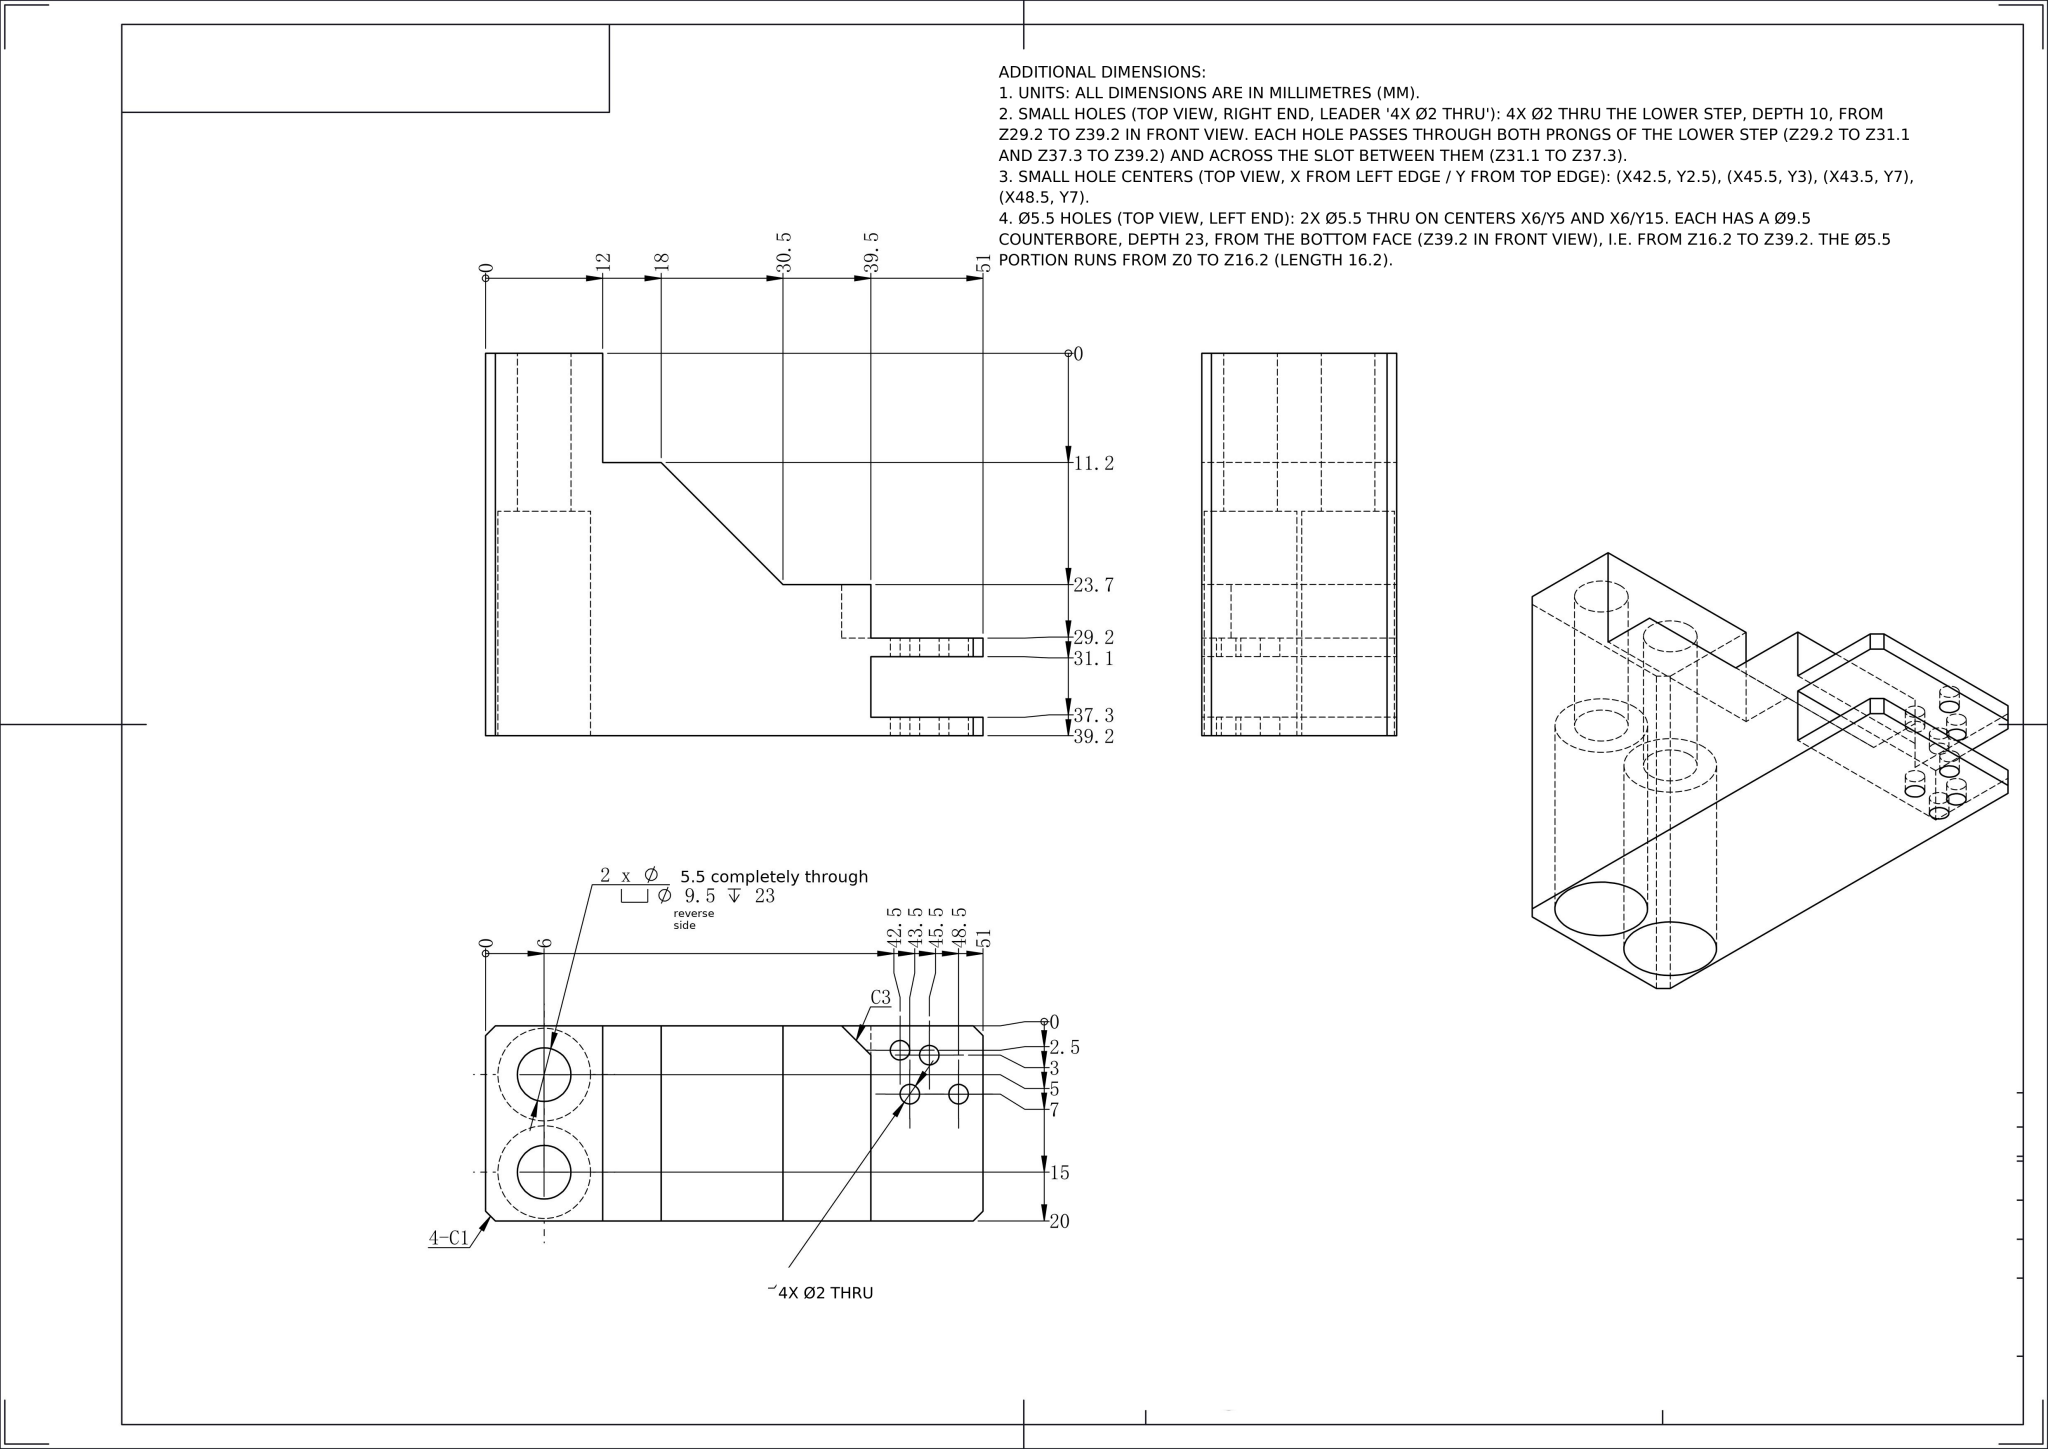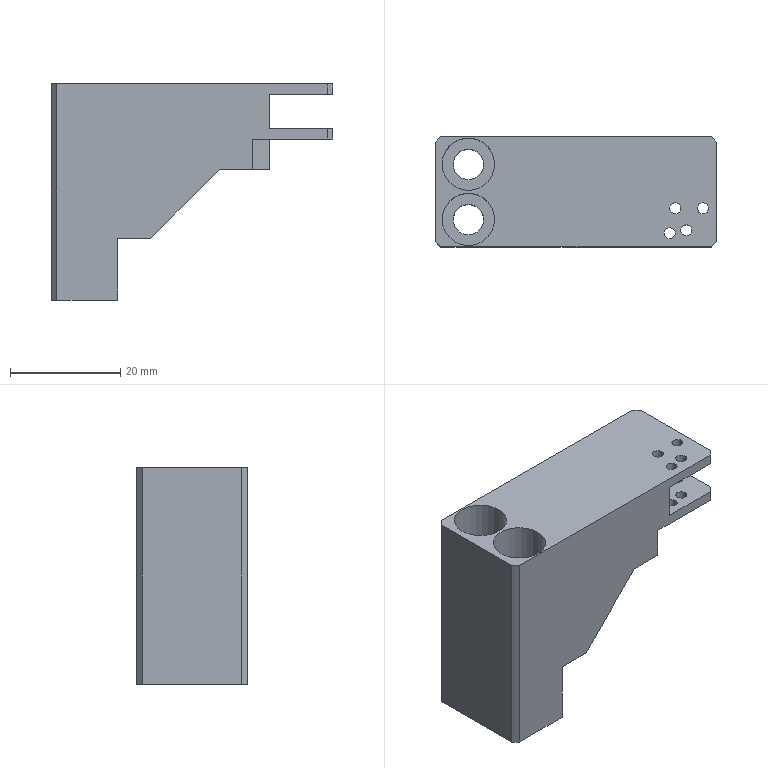Part | NX | mm | 1 solid | 49 faces | box 51 x 20 x 39.2 mm | volume 17724 mm3 | plane 25 | cylinder 24 | commonest cylinder face diameters 2 x16 9.5 x4 5.5 x4